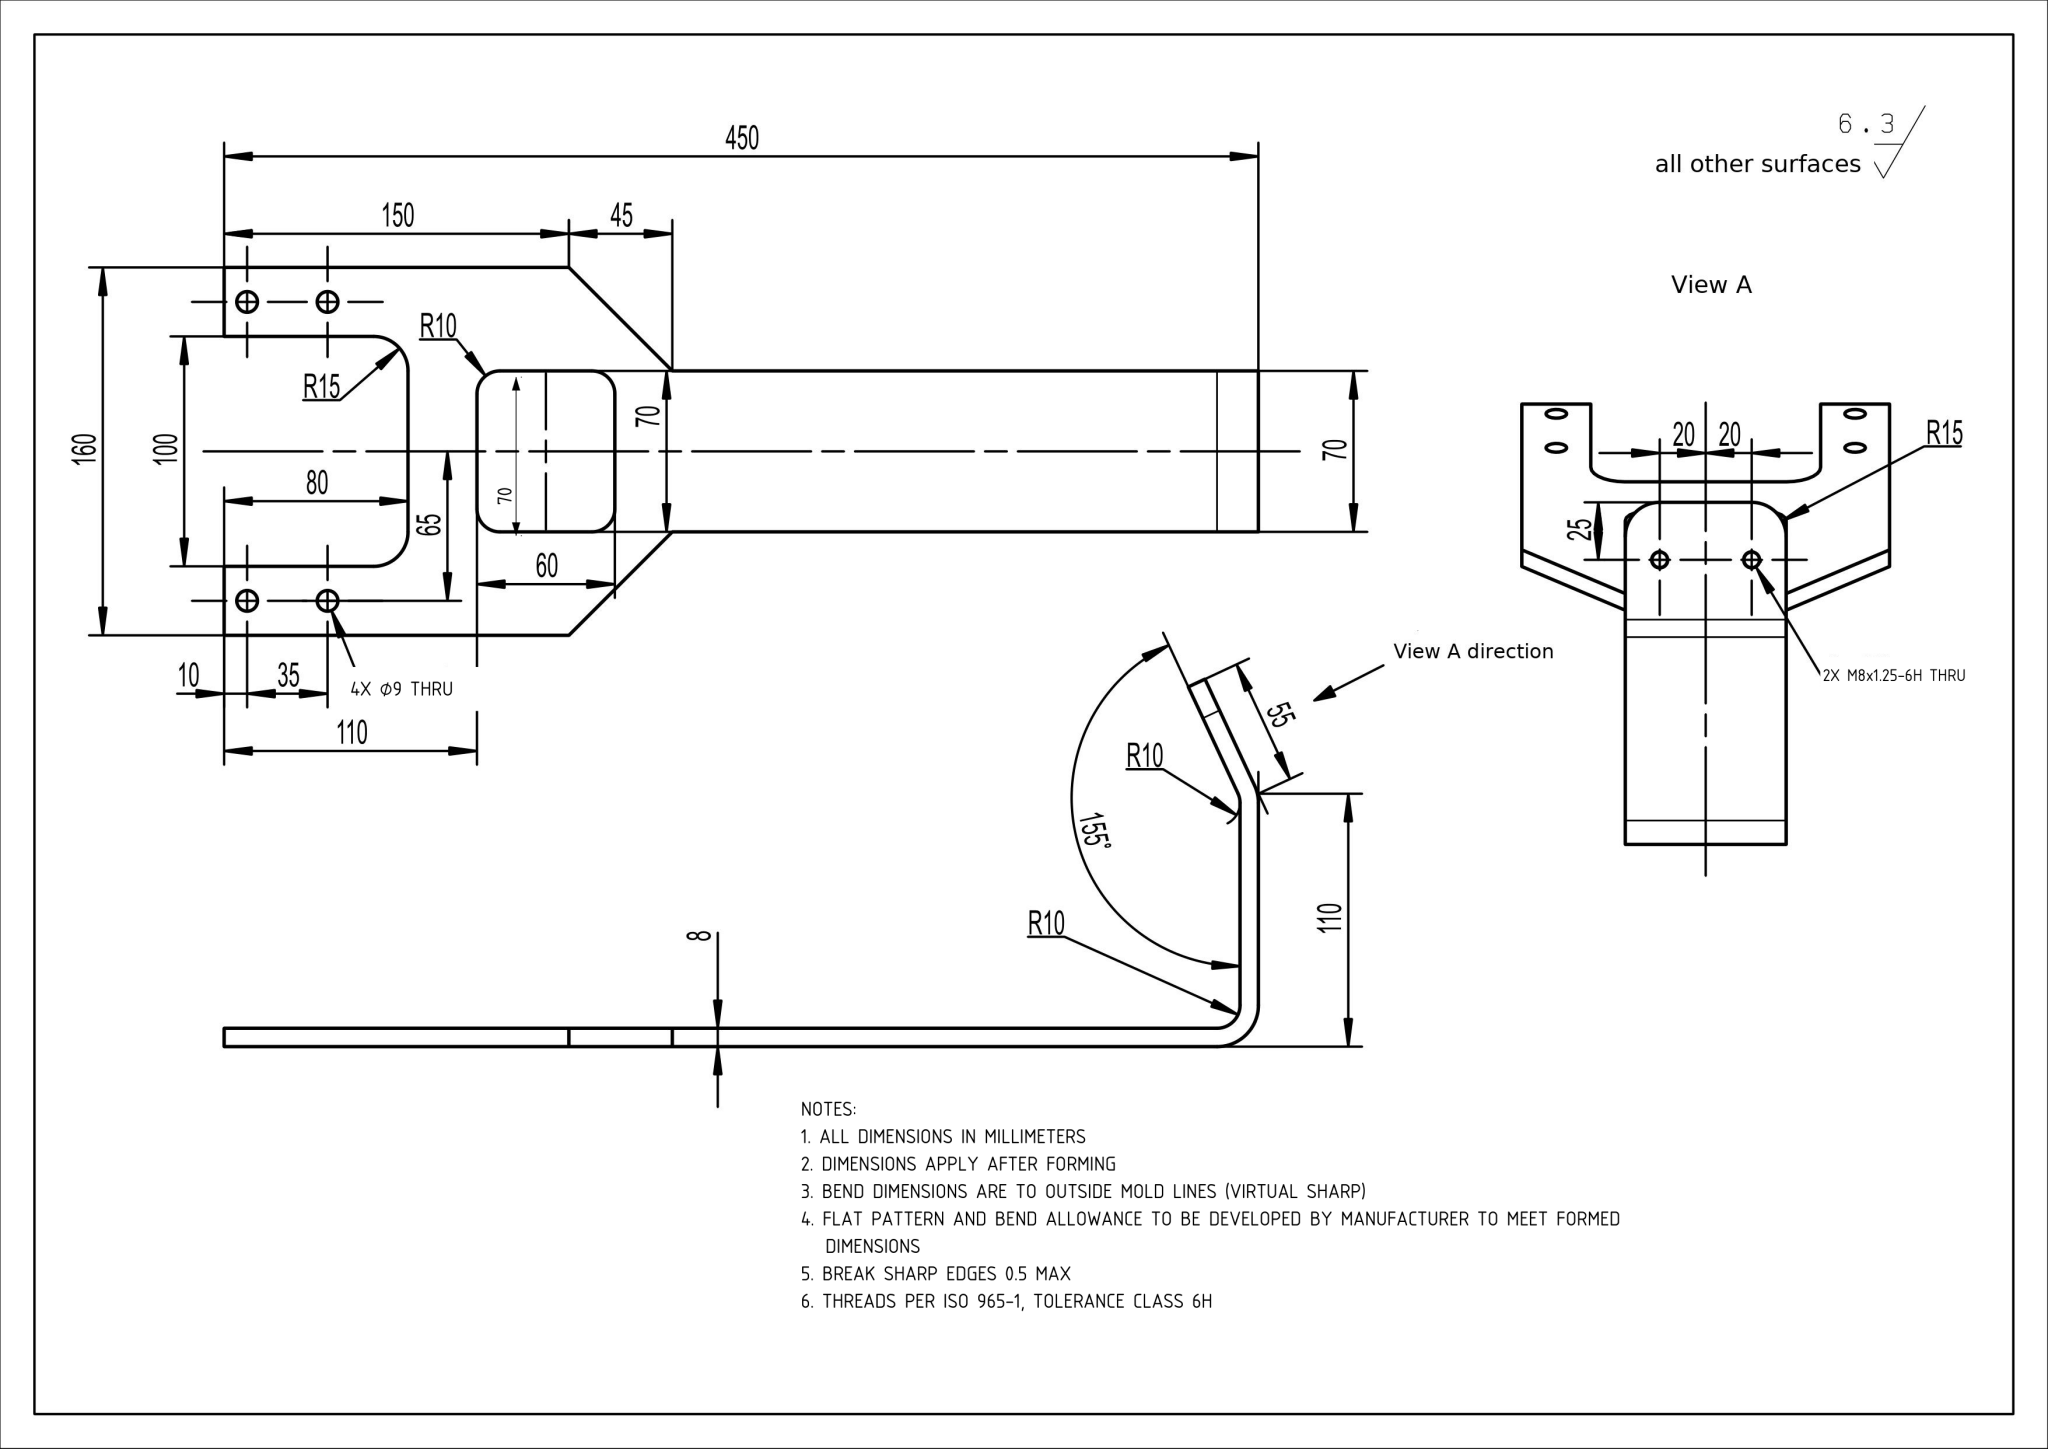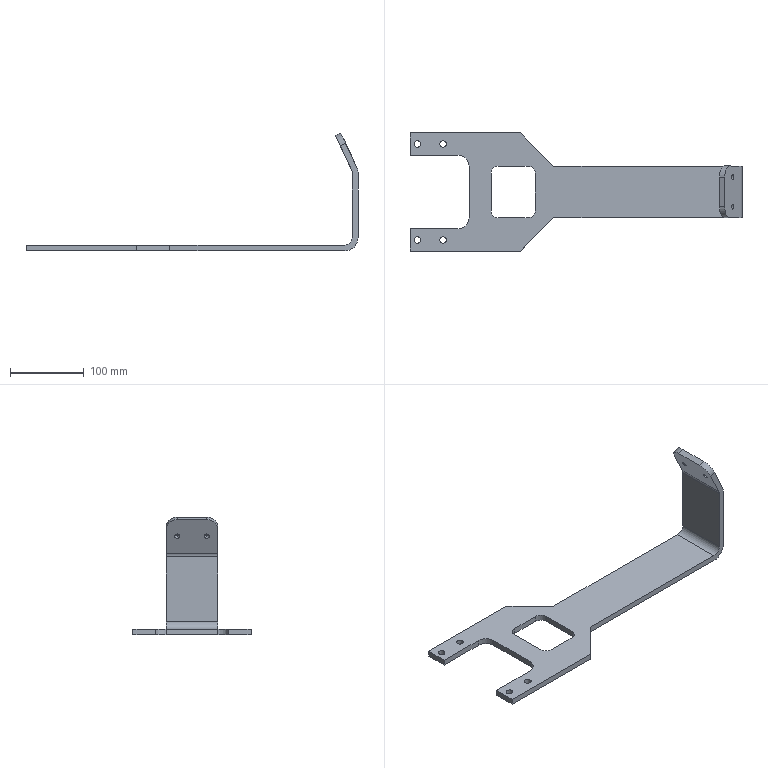Part | NX | mm | 1 solid | 40 faces | box 450 x 160 x 159.85 mm | volume 360176 mm3 | plane 22 | cylinder 18 | commonest cylinder face diameters 20 x6 9 x4 30 x4 36 x2 6.8 x2